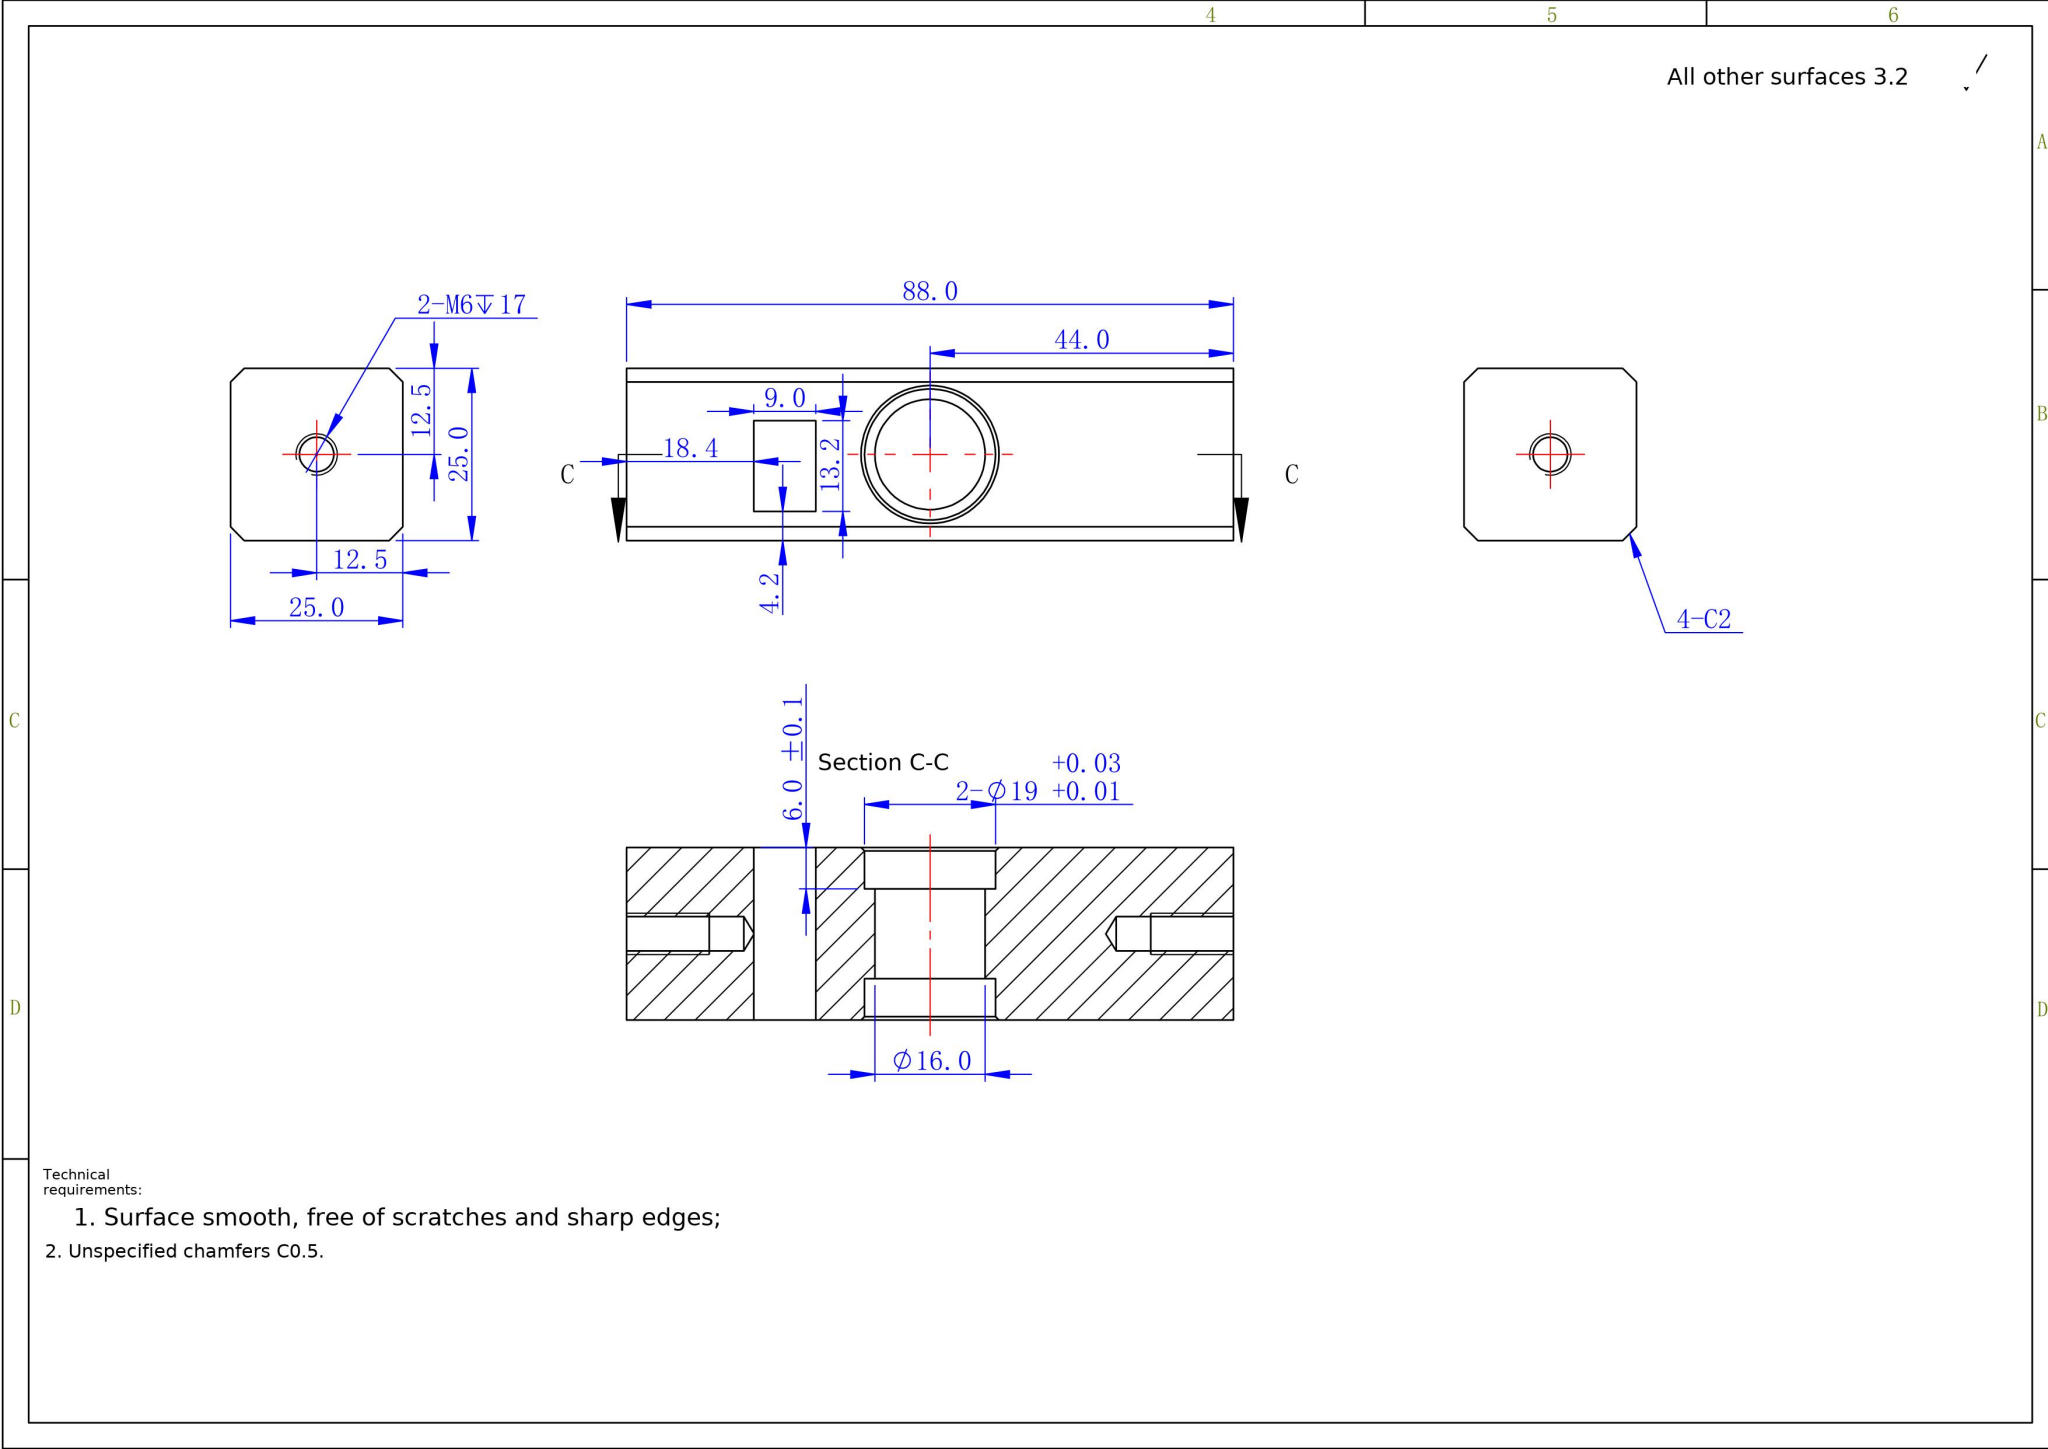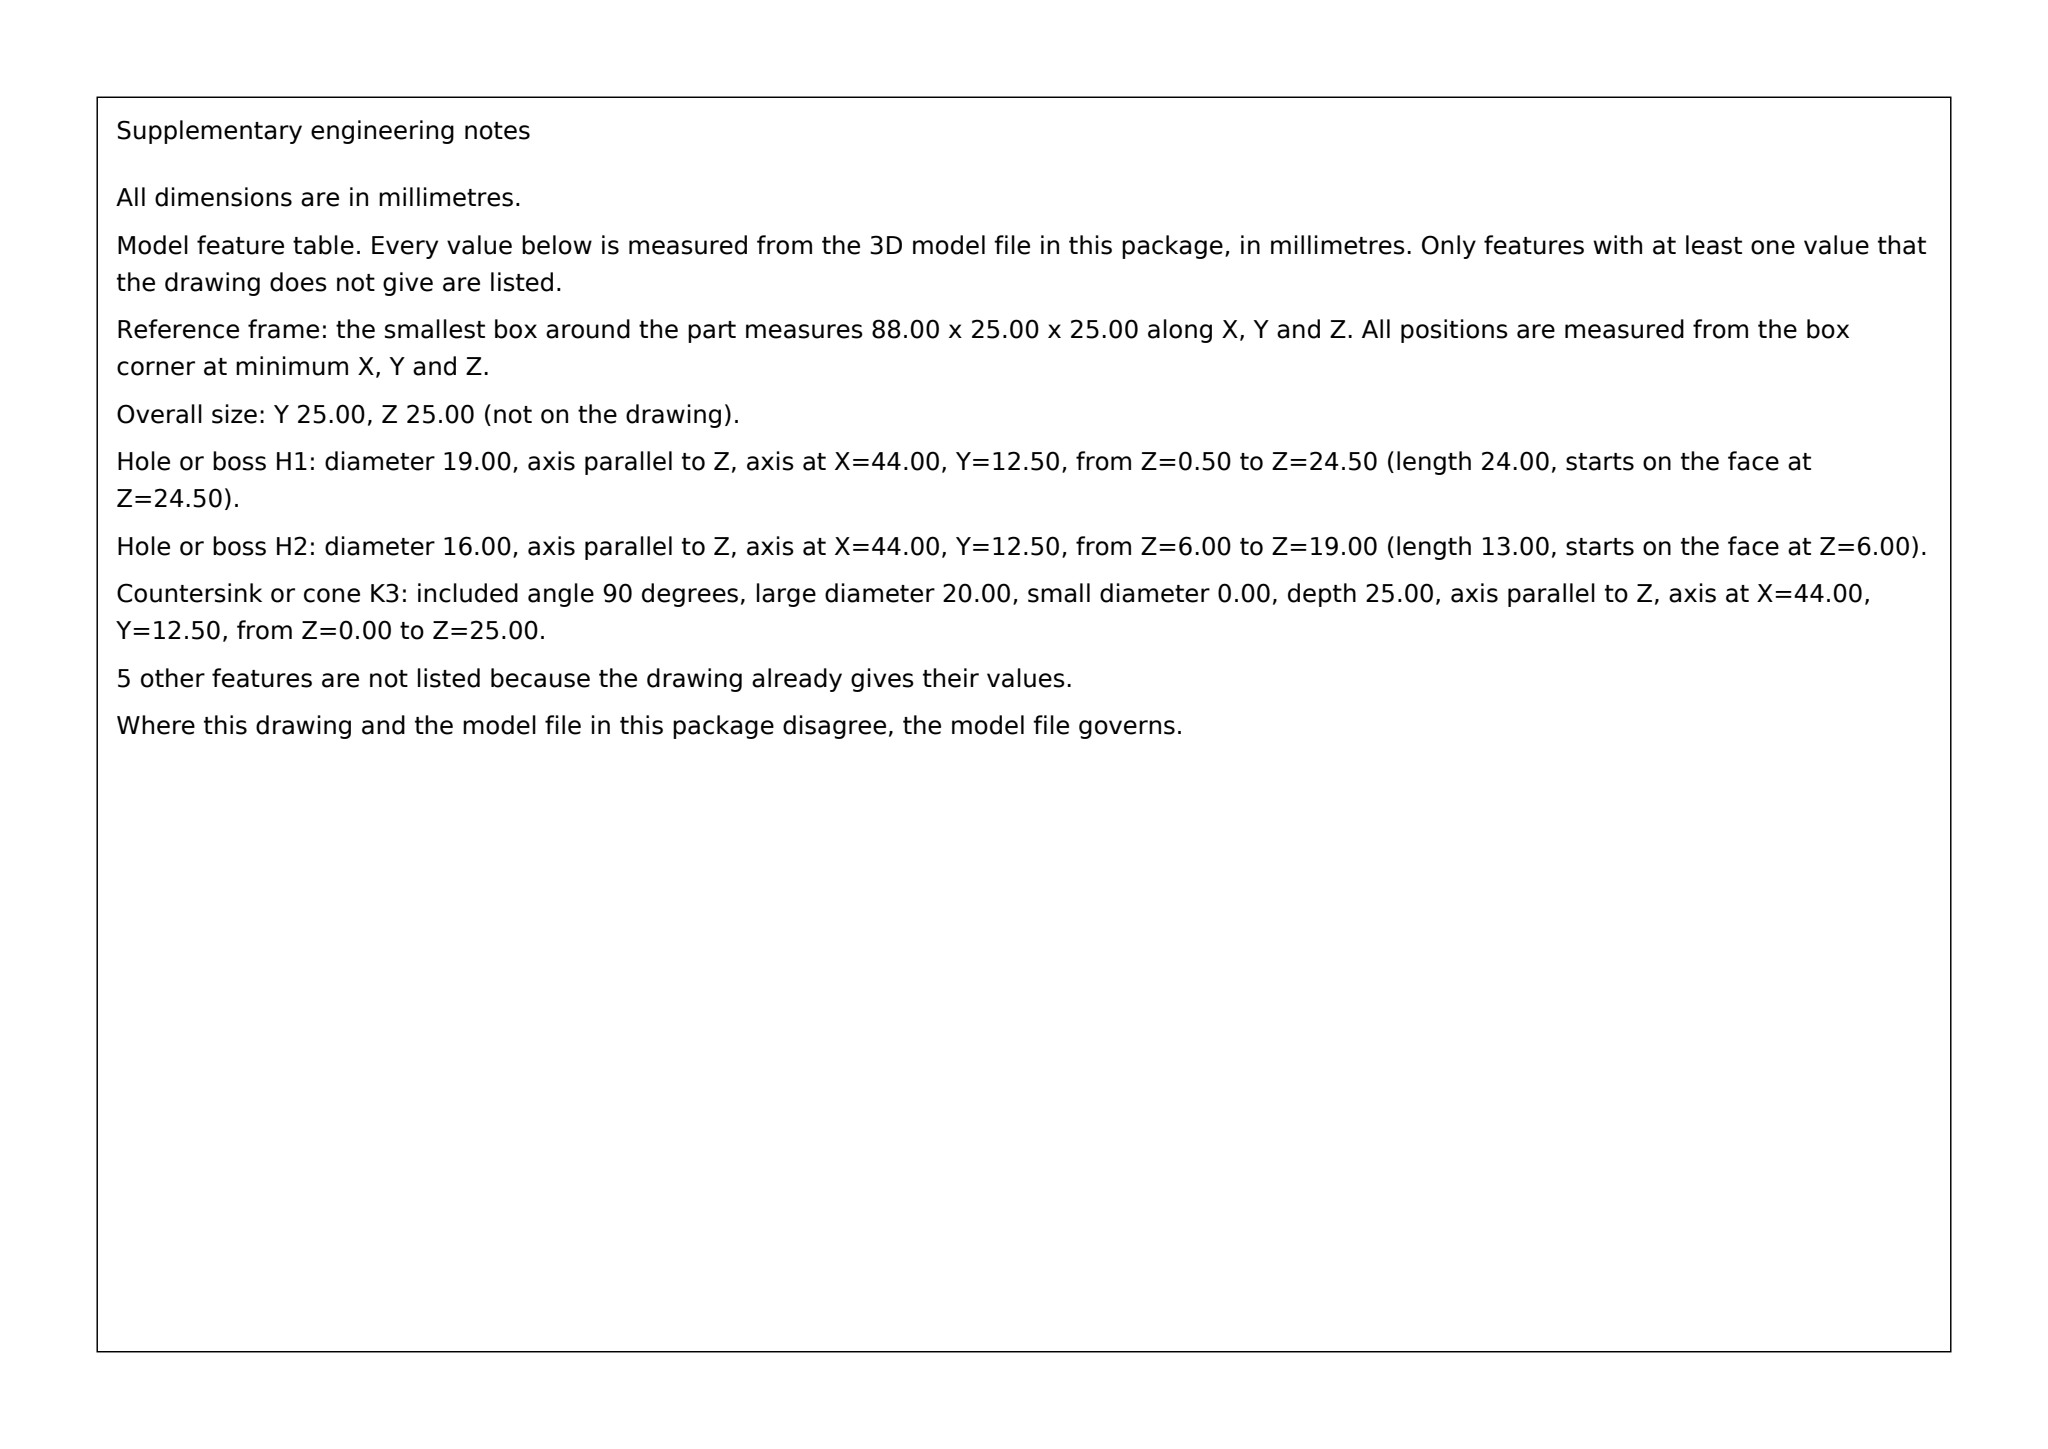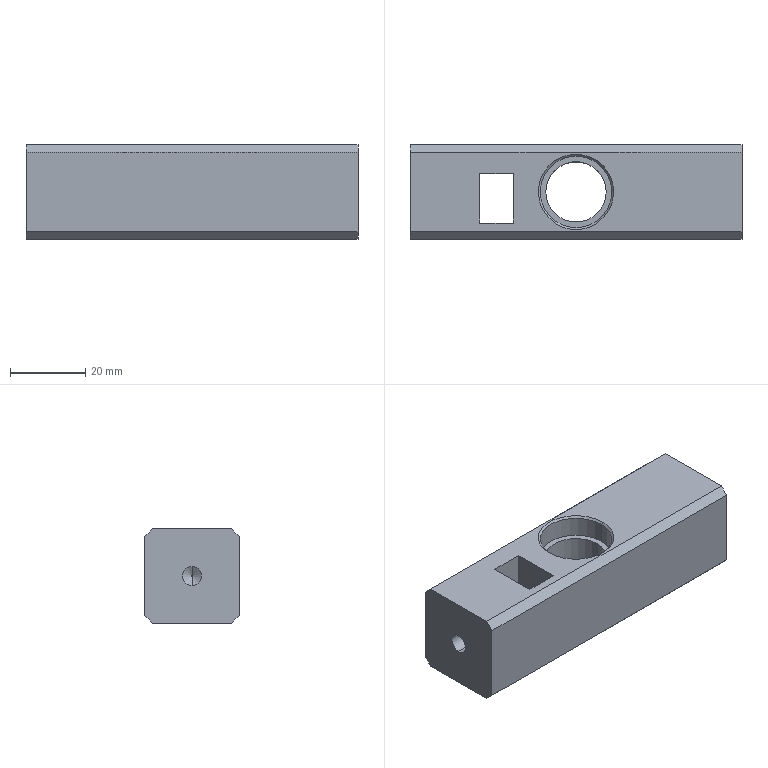Part | SolidWorks | mm | 1 solid | 34 faces | box 88 x 25 x 25 mm | volume 44622 mm3 | plane 16 | cylinder 10 | cone 8 | commonest cylinder face diameters 5 x4 19 x4 16 x2